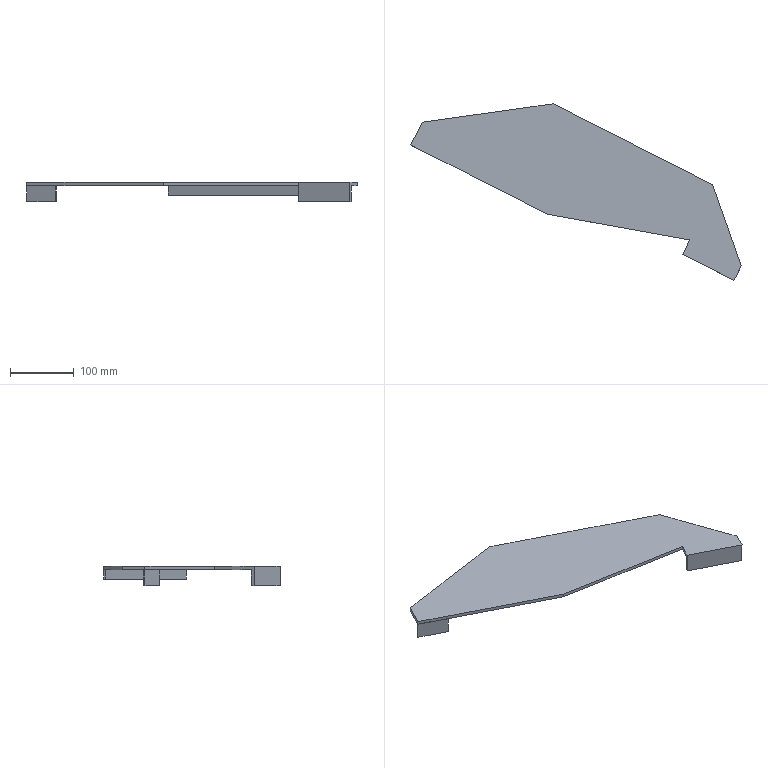Component | SolidWorks | Part17-1 | 2 solids | 23 faces | box 517.58 x 276.19 x 30 mm | volume 334372 mm3 | plane 23
build123d program:
from build123d import *

# Parameters (mm, degrees)
SKETCH1_W           = 90
SKETCH1_H           = 30
BOSS_EXTRUDE1_DEPTH = 5
BOSS_EXTRUDE2_DEPTH = 5
SKETCH3_W           = 280
SKETCH3_H           = 15
BOSS_EXTRUDE7_DEPTH = 3
BOSS_EXTRUDE8_DEPTH = 3


with BuildPart() as part:
    # Sketch1 → Boss-Extrude1 (new body)
    with BuildSketch(Plane.XY):
        with Locations((-7.063, 15)):
            Rectangle(SKETCH1_W, SKETCH1_H)
    extrude(amount=BOSS_EXTRUDE1_DEPTH)

    # Sketch2 → Boss-Extrude2 (add)
    with BuildSketch(Plane(origin=(0, 30, 0), x_dir=(-1, 0, 0), z_dir=(0, -1, 0))):
        Polygon((-37.937, 0), (-37.937, 20), (59.702, 113.229), (339.702, 113.229), (509.386, -5), (509.386, -45), (269.386, -45), (52.063, 20), (52.063, 0), (52.063, -5), (-37.937, -5), align=None)
    extrude(amount=BOSS_EXTRUDE2_DEPTH)

    # Sketch3 → Boss-Extrude7 (add)
    with BuildSketch(Plane(origin=(0, 0, -113.229), x_dir=(-1, 0, 0), z_dir=(0, 0, -1))):
        with Locations((199.702, 17.5)):
            Rectangle(SKETCH3_W, SKETCH3_H)
    extrude(amount=-BOSS_EXTRUDE7_DEPTH)


with BuildPart() as body_2:
    # Sketch6 → Boss-Extrude8 (new body)
    with BuildSketch(Plane.XY.offset(45)):
        Polygon((-509.386, 25), (-509.386, 0), (-459.386, 0), (-459.386, 24.804), align=None)
    extrude(amount=-BOSS_EXTRUDE8_DEPTH)


solid = Compound([part.part, body_2.part])

# Placed as in the assembly
solid = solid.moved(Location((298.812, -1061.476, 2432.971), (90, -26.879, 0)))
STEP:
#1=COLOUR_RGB('',0.7922,0.8196,0.9333);
#2=FILL_AREA_STYLE_COLOUR('',#1);
#3=FILL_AREA_STYLE('',(#2));
#4=SURFACE_STYLE_FILL_AREA(#3);
#5=SURFACE_SIDE_STYLE('',(#4));
#6=SURFACE_STYLE_USAGE(.BOTH.,#5);
#7=PRESENTATION_STYLE_ASSIGNMENT((#6));
#8=CARTESIAN_POINT('',(-6.213,-32.899,96.771));
#9=VERTEX_POINT('',#8);
#10=CARTESIAN_POINT('',(1.85,-31.768,96.771));
#11=VERTEX_POINT('',#10);
#12=CARTESIAN_POINT('',(-6.213,-32.899,96.771));
#13=DIRECTION('',(0.9903,0.139,0.));
#14=VECTOR('',#13,39.37);
#15=LINE('',#12,#14);
#16=EDGE_CURVE('',#9,#11,#15,.T.);
#17=ORIENTED_EDGE('',*,*,#16,.T.);
#18=CARTESIAN_POINT('',(1.797,-31.873,96.771));
#19=VERTEX_POINT('',#18);
#20=CARTESIAN_POINT('',(1.797,-31.873,96.771));
#21=DIRECTION('',(0.4521,0.892,0.));
#22=VECTOR('',#21,39.37);
#23=LINE('',#20,#22);
#24=EDGE_CURVE('',#19,#11,#23,.T.);
#25=ORIENTED_EDGE('',*,*,#24,.F.);
#26=CARTESIAN_POINT('',(11.63,-36.857,96.771));
#27=VERTEX_POINT('',#26);
#28=CARTESIAN_POINT('',(11.63,-36.857,96.771));
#29=DIRECTION('',(-0.892,0.4521,0.));
#30=VECTOR('',#29,39.37);
#31=LINE('',#28,#30);
#32=EDGE_CURVE('',#27,#19,#31,.T.);
#33=ORIENTED_EDGE('',*,*,#32,.F.);
#34=CARTESIAN_POINT('',(11.683,-36.751,96.771));
#35=VERTEX_POINT('',#34);
#36=CARTESIAN_POINT('',(11.63,-36.857,96.771));
#37=DIRECTION('',(0.4521,0.892,0.));
#38=VECTOR('',#37,39.37);
#39=LINE('',#36,#38);
#40=EDGE_CURVE('',#27,#35,#39,.T.);
#41=ORIENTED_EDGE('',*,*,#40,.T.);
#42=CARTESIAN_POINT('',(13.452,-41.763,96.771));
#43=VERTEX_POINT('',#42);
#44=CARTESIAN_POINT('',(13.452,-41.763,96.771));
#45=DIRECTION('',(0.3329,-0.943,-0.));
#46=VECTOR('',#45,39.37);
#47=LINE('',#44,#46);
#48=EDGE_CURVE('',#35,#43,#47,.T.);
#49=ORIENTED_EDGE('',*,*,#48,.T.);
#50=CARTESIAN_POINT('',(13.096,-42.466,96.771));
#51=VERTEX_POINT('',#50);
#52=CARTESIAN_POINT('',(13.096,-42.466,96.771));
#53=DIRECTION('',(-0.4521,-0.892,-0.));
#54=VECTOR('',#53,39.37);
#55=LINE('',#52,#54);
#56=EDGE_CURVE('',#43,#51,#55,.T.);
#57=ORIENTED_EDGE('',*,*,#56,.T.);
#58=CARTESIAN_POINT('',(9.936,-40.864,96.771));
#59=VERTEX_POINT('',#58);
#60=CARTESIAN_POINT('',(11.764,-41.79,96.771));
#61=DIRECTION('',(0.892,-0.4521,-0.));
#62=VECTOR('',#61,39.37);
#63=LINE('',#60,#62);
#64=EDGE_CURVE('',#59,#51,#63,.T.);
#65=ORIENTED_EDGE('',*,*,#64,.F.);
#66=CARTESIAN_POINT('',(10.292,-40.161,96.771));
#67=VERTEX_POINT('',#66);
#68=CARTESIAN_POINT('',(9.847,-41.039,96.771));
#69=DIRECTION('',(0.4521,0.892,0.));
#70=VECTOR('',#69,39.37);
#71=LINE('',#68,#70);
#72=EDGE_CURVE('',#59,#67,#71,.T.);
#73=ORIENTED_EDGE('',*,*,#72,.T.);
#74=CARTESIAN_POINT('',(1.503,-38.576,96.771));
#75=VERTEX_POINT('',#74);
#76=CARTESIAN_POINT('',(10.292,-40.161,96.771));
#77=DIRECTION('',(-0.9841,0.1775,0.));
#78=VECTOR('',#77,39.37);
#79=LINE('',#76,#78);
#80=EDGE_CURVE('',#67,#75,#79,.T.);
#81=ORIENTED_EDGE('',*,*,#80,.T.);
#82=CARTESIAN_POINT('',(-6.925,-34.304,96.771));
#83=VERTEX_POINT('',#82);
#84=CARTESIAN_POINT('',(1.503,-38.576,96.771));
#85=DIRECTION('',(-0.892,0.4521,0.));
#86=VECTOR('',#85,39.37);
#87=LINE('',#84,#86);
#88=EDGE_CURVE('',#75,#83,#87,.T.);
#89=ORIENTED_EDGE('',*,*,#88,.T.);
#90=CARTESIAN_POINT('',(-6.925,-34.304,96.771));
#91=DIRECTION('',(0.4521,0.892,0.));
#92=VECTOR('',#91,39.37);
#93=LINE('',#90,#92);
#94=EDGE_CURVE('',#83,#9,#93,.T.);
#95=ORIENTED_EDGE('',*,*,#94,.T.);
#96=EDGE_LOOP('',(#17,#25,#33,#41,#49,#57,#65,#73,#81,#89,#95));
#97=FACE_OUTER_BOUND('',#96,.T.);
#98=CARTESIAN_POINT('',(11.764,-41.79,96.771));
#99=DIRECTION('',(0.,0.,-1.));
#100=DIRECTION('',(0.4521,0.892,0.));
#101=AXIS2_PLACEMENT_3D('',#98,#99,#100);
#102=PLANE('',#101);
#103=ADVANCED_FACE('',(#97),#102,.T.);
#104=CARTESIAN_POINT('',(9.847,-41.039,95.786));
#105=VERTEX_POINT('',#104);
#106=CARTESIAN_POINT('',(9.936,-40.864,95.786));
#107=VERTEX_POINT('',#106);
#108=CARTESIAN_POINT('',(9.847,-41.039,95.786));
#109=DIRECTION('',(0.4521,0.892,0.));
#110=VECTOR('',#109,39.37);
#111=LINE('',#108,#110);
#112=EDGE_CURVE('',#105,#107,#111,.T.);
#113=ORIENTED_EDGE('',*,*,#112,.F.);
#114=CARTESIAN_POINT('',(9.847,-41.039,96.967));
#115=VERTEX_POINT('',#114);
#116=CARTESIAN_POINT('',(9.847,-41.039,96.967));
#117=DIRECTION('',(0.,0.,-1.));
#118=VECTOR('',#117,39.37);
#119=LINE('',#116,#118);
#120=EDGE_CURVE('',#115,#105,#119,.T.);
#121=ORIENTED_EDGE('',*,*,#120,.F.);
#122=CARTESIAN_POINT('',(10.292,-40.161,96.967));
#123=VERTEX_POINT('',#122);
#124=CARTESIAN_POINT('',(9.847,-41.039,96.967));
#125=DIRECTION('',(0.4521,0.892,0.));
#126=VECTOR('',#125,39.37);
#127=LINE('',#124,#126);
#128=EDGE_CURVE('',#115,#123,#127,.T.);
#129=ORIENTED_EDGE('',*,*,#128,.T.);
#130=CARTESIAN_POINT('',(10.292,-40.161,96.771));
#131=DIRECTION('',(-0.,-0.,1.));
#132=VECTOR('',#131,39.37);
#133=LINE('',#130,#132);
#134=EDGE_CURVE('',#67,#123,#133,.T.);
#135=ORIENTED_EDGE('',*,*,#134,.F.);
#136=ORIENTED_EDGE('',*,*,#72,.F.);
#137=CARTESIAN_POINT('',(9.936,-40.864,96.967));
#138=DIRECTION('',(0.,0.,-1.));
#139=VECTOR('',#138,39.37);
#140=LINE('',#137,#139);
#141=EDGE_CURVE('',#59,#107,#140,.T.);
#142=ORIENTED_EDGE('',*,*,#141,.T.);
#143=EDGE_LOOP('',(#113,#121,#129,#135,#136,#142));
#144=FACE_OUTER_BOUND('',#143,.T.);
#145=CARTESIAN_POINT('',(9.847,-41.039,96.967));
#146=DIRECTION('',(0.892,-0.4521,-0.));
#147=DIRECTION('',(0.4521,0.892,0.));
#148=AXIS2_PLACEMENT_3D('',#145,#146,#147);
#149=PLANE('',#148);
#150=ADVANCED_FACE('',(#144),#149,.F.);
#151=CARTESIAN_POINT('',(13.096,-42.466,95.786));
#152=VERTEX_POINT('',#151);
#153=CARTESIAN_POINT('',(9.936,-40.864,95.786));
#154=DIRECTION('',(0.892,-0.4521,-0.));
#155=VECTOR('',#154,39.37);
#156=LINE('',#153,#155);
#157=EDGE_CURVE('',#107,#152,#156,.T.);
#158=ORIENTED_EDGE('',*,*,#157,.T.);
#159=CARTESIAN_POINT('',(13.007,-42.641,95.786));
#160=VERTEX_POINT('',#159);
#161=CARTESIAN_POINT('',(13.007,-42.641,95.786));
#162=DIRECTION('',(0.4521,0.892,0.));
#163=VECTOR('',#162,39.37);
#164=LINE('',#161,#163);
#165=EDGE_CURVE('',#160,#152,#164,.T.);
#166=ORIENTED_EDGE('',*,*,#165,.F.);
#167=CARTESIAN_POINT('',(9.847,-41.039,95.786));
#168=DIRECTION('',(0.892,-0.4521,-0.));
#169=VECTOR('',#168,39.37);
#170=LINE('',#167,#169);
#171=EDGE_CURVE('',#105,#160,#170,.T.);
#172=ORIENTED_EDGE('',*,*,#171,.F.);
#173=ORIENTED_EDGE('',*,*,#112,.T.);
#174=EDGE_LOOP('',(#158,#166,#172,#173));
#175=FACE_OUTER_BOUND('',#174,.T.);
#176=CARTESIAN_POINT('',(9.847,-41.039,95.786));
#177=DIRECTION('',(-0.,-0.,1.));
#178=DIRECTION('',(-0.4521,-0.892,-0.));
#179=AXIS2_PLACEMENT_3D('',#176,#177,#178);
#180=PLANE('',#179);
#181=ADVANCED_FACE('',(#175),#180,.F.);
#182=CARTESIAN_POINT('',(13.096,-42.466,96.967));
#183=DIRECTION('',(-0.,-0.,1.));
#184=VECTOR('',#183,39.37);
#185=LINE('',#182,#184);
#186=EDGE_CURVE('',#152,#51,#185,.T.);
#187=ORIENTED_EDGE('',*,*,#186,.T.);
#188=ORIENTED_EDGE('',*,*,#56,.F.);
#189=CARTESIAN_POINT('',(13.452,-41.763,96.967));
#190=VERTEX_POINT('',#189);
#191=CARTESIAN_POINT('',(13.452,-41.763,96.771));
#192=DIRECTION('',(-0.,-0.,1.));
#193=VECTOR('',#192,39.37);
#194=LINE('',#191,#193);
#195=EDGE_CURVE('',#43,#190,#194,.T.);
#196=ORIENTED_EDGE('',*,*,#195,.T.);
#197=CARTESIAN_POINT('',(13.007,-42.641,96.967));
#198=VERTEX_POINT('',#197);
#199=CARTESIAN_POINT('',(13.007,-42.641,96.967));
#200=DIRECTION('',(0.4521,0.892,0.));
#201=VECTOR('',#200,39.37);
#202=LINE('',#199,#201);
#203=EDGE_CURVE('',#198,#190,#202,.T.);
#204=ORIENTED_EDGE('',*,*,#203,.F.);
#205=CARTESIAN_POINT('',(13.007,-42.641,96.967));
#206=DIRECTION('',(-0.,-0.,1.));
#207=VECTOR('',#206,39.37);
#208=LINE('',#205,#207);
#209=EDGE_CURVE('',#160,#198,#208,.T.);
#210=ORIENTED_EDGE('',*,*,#209,.F.);
#211=ORIENTED_EDGE('',*,*,#165,.T.);
#212=EDGE_LOOP('',(#187,#188,#196,#204,#210,#211));
#213=FACE_OUTER_BOUND('',#212,.T.);
#214=CARTESIAN_POINT('',(13.007,-42.641,96.967));
#215=DIRECTION('',(-0.892,0.4521,0.));
#216=DIRECTION('',(-0.4521,-0.892,-0.));
#217=AXIS2_PLACEMENT_3D('',#214,#215,#216);
#218=PLANE('',#217);
#219=ADVANCED_FACE('',(#213),#218,.F.);
#220=ORIENTED_EDGE('',*,*,#203,.T.);
#221=CARTESIAN_POINT('',(11.683,-36.751,96.967));
#222=VERTEX_POINT('',#221);
#223=CARTESIAN_POINT('',(13.452,-41.763,96.967));
#224=DIRECTION('',(0.3329,-0.943,-0.));
#225=VECTOR('',#224,39.37);
#226=LINE('',#223,#225);
#227=EDGE_CURVE('',#222,#190,#226,.T.);
#228=ORIENTED_EDGE('',*,*,#227,.F.);
#229=CARTESIAN_POINT('',(1.85,-31.768,96.967));
#230=VERTEX_POINT('',#229);
#231=CARTESIAN_POINT('',(11.683,-36.751,96.967));
#232=DIRECTION('',(0.892,-0.4521,-0.));
#233=VECTOR('',#232,39.37);
#234=LINE('',#231,#233);
#235=EDGE_CURVE('',#230,#222,#234,.T.);
#236=ORIENTED_EDGE('',*,*,#235,.F.);
#237=CARTESIAN_POINT('',(-6.213,-32.899,96.967));
#238=VERTEX_POINT('',#237);
#239=CARTESIAN_POINT('',(-6.213,-32.899,96.967));
#240=DIRECTION('',(0.9903,0.139,0.));
#241=VECTOR('',#240,39.37);
#242=LINE('',#239,#241);
#243=EDGE_CURVE('',#238,#230,#242,.T.);
#244=ORIENTED_EDGE('',*,*,#243,.F.);
#245=CARTESIAN_POINT('',(-6.925,-34.304,96.967));
#246=VERTEX_POINT('',#245);
#247=CARTESIAN_POINT('',(-6.925,-34.304,96.967));
#248=DIRECTION('',(0.4521,0.892,0.));
#249=VECTOR('',#248,39.37);
#250=LINE('',#247,#249);
#251=EDGE_CURVE('',#246,#238,#250,.T.);
#252=ORIENTED_EDGE('',*,*,#251,.F.);
#253=CARTESIAN_POINT('',(1.503,-38.576,96.967));
#254=VERTEX_POINT('',#253);
#255=CARTESIAN_POINT('',(1.503,-38.576,96.967));
#256=DIRECTION('',(-0.892,0.4521,0.));
#257=VECTOR('',#256,39.37);
#258=LINE('',#255,#257);
#259=EDGE_CURVE('',#254,#246,#258,.T.);
#260=ORIENTED_EDGE('',*,*,#259,.F.);
#261=CARTESIAN_POINT('',(10.292,-40.161,96.967));
#262=DIRECTION('',(-0.9841,0.1775,0.));
#263=VECTOR('',#262,39.37);
#264=LINE('',#261,#263);
#265=EDGE_CURVE('',#123,#254,#264,.T.);
#266=ORIENTED_EDGE('',*,*,#265,.F.);
#267=ORIENTED_EDGE('',*,*,#128,.F.);
#268=CARTESIAN_POINT('',(9.847,-41.039,96.967));
#269=DIRECTION('',(-0.892,0.4521,0.));
#270=VECTOR('',#269,39.37);
#271=LINE('',#268,#270);
#272=EDGE_CURVE('',#198,#115,#271,.T.);
#273=ORIENTED_EDGE('',*,*,#272,.F.);
#274=EDGE_LOOP('',(#220,#228,#236,#244,#252,#260,#266,#267,#273));
#275=FACE_OUTER_BOUND('',#274,.T.);
#276=CARTESIAN_POINT('',(9.847,-41.039,96.967));
#277=DIRECTION('',(0.,0.,-1.));
#278=DIRECTION('',(0.4521,0.892,0.));
#279=AXIS2_PLACEMENT_3D('',#276,#277,#278);
#280=PLANE('',#279);
#281=ADVANCED_FACE('',(#275),#280,.F.);
#282=ORIENTED_EDGE('',*,*,#209,.T.);
#283=ORIENTED_EDGE('',*,*,#272,.T.);
#284=ORIENTED_EDGE('',*,*,#120,.T.);
#285=ORIENTED_EDGE('',*,*,#171,.T.);
#286=EDGE_LOOP('',(#282,#283,#284,#285));
#287=FACE_OUTER_BOUND('',#286,.T.);
#288=CARTESIAN_POINT('',(11.675,-41.966,95.786));
#289=DIRECTION('',(-0.4521,-0.892,-0.));
#290=DIRECTION('',(0.892,-0.4521,-0.));
#291=AXIS2_PLACEMENT_3D('',#288,#289,#290);
#292=PLANE('',#291);
#293=ADVANCED_FACE('',(#287),#292,.T.);
#294=ORIENTED_EDGE('',*,*,#141,.F.);
#295=ORIENTED_EDGE('',*,*,#64,.T.);
#296=ORIENTED_EDGE('',*,*,#186,.F.);
#297=ORIENTED_EDGE('',*,*,#157,.F.);
#298=EDGE_LOOP('',(#294,#295,#296,#297));
#299=FACE_OUTER_BOUND('',#298,.T.);
#300=CARTESIAN_POINT('',(11.764,-41.79,95.786));
#301=DIRECTION('',(-0.4521,-0.892,-0.));
#302=DIRECTION('',(0.892,-0.4521,-0.));
#303=AXIS2_PLACEMENT_3D('',#300,#301,#302);
#304=PLANE('',#303);
#305=ADVANCED_FACE('',(#299),#304,.F.);
#306=ORIENTED_EDGE('',*,*,#265,.T.);
#307=CARTESIAN_POINT('',(1.503,-38.576,96.771));
#308=DIRECTION('',(-0.,-0.,1.));
#309=VECTOR('',#308,39.37);
#310=LINE('',#307,#309);
#311=EDGE_CURVE('',#75,#254,#310,.T.);
#312=ORIENTED_EDGE('',*,*,#311,.F.);
#313=ORIENTED_EDGE('',*,*,#80,.F.);
#314=ORIENTED_EDGE('',*,*,#134,.T.);
#315=EDGE_LOOP('',(#306,#312,#313,#314));
#316=FACE_OUTER_BOUND('',#315,.T.);
#317=CARTESIAN_POINT('',(10.292,-40.161,96.771));
#318=DIRECTION('',(0.1775,0.9841,0.));
#319=DIRECTION('',(-0.9841,0.1775,0.));
#320=AXIS2_PLACEMENT_3D('',#317,#318,#319);
#321=PLANE('',#320);
#322=ADVANCED_FACE('',(#316),#321,.F.);
#323=ORIENTED_EDGE('',*,*,#259,.T.);
#324=CARTESIAN_POINT('',(-6.925,-34.304,96.771));
#325=DIRECTION('',(-0.,-0.,1.));
#326=VECTOR('',#325,39.37);
#327=LINE('',#324,#326);
#328=EDGE_CURVE('',#83,#246,#327,.T.);
#329=ORIENTED_EDGE('',*,*,#328,.F.);
#330=ORIENTED_EDGE('',*,*,#88,.F.);
#331=ORIENTED_EDGE('',*,*,#311,.T.);
#332=EDGE_LOOP('',(#323,#329,#330,#331));
#333=FACE_OUTER_BOUND('',#332,.T.);
#334=CARTESIAN_POINT('',(1.503,-38.576,96.771));
#335=DIRECTION('',(0.4521,0.892,0.));
#336=DIRECTION('',(-0.892,0.4521,0.));
#337=AXIS2_PLACEMENT_3D('',#334,#335,#336);
#338=PLANE('',#337);
#339=ADVANCED_FACE('',(#333),#338,.F.);
#340=ORIENTED_EDGE('',*,*,#251,.T.);
#341=CARTESIAN_POINT('',(-6.213,-32.899,96.771));
#342=DIRECTION('',(-0.,-0.,1.));
#343=VECTOR('',#342,39.37);
#344=LINE('',#341,#343);
#345=EDGE_CURVE('',#9,#238,#344,.T.);
#346=ORIENTED_EDGE('',*,*,#345,.F.);
#347=ORIENTED_EDGE('',*,*,#94,.F.);
#348=ORIENTED_EDGE('',*,*,#328,.T.);
#349=EDGE_LOOP('',(#340,#346,#347,#348));
#350=FACE_OUTER_BOUND('',#349,.T.);
#351=CARTESIAN_POINT('',(-6.925,-34.304,96.771));
#352=DIRECTION('',(0.892,-0.4521,-0.));
#353=DIRECTION('',(0.4521,0.892,0.));
#354=AXIS2_PLACEMENT_3D('',#351,#352,#353);
#355=PLANE('',#354);
#356=ADVANCED_FACE('',(#350),#355,.F.);
#357=ORIENTED_EDGE('',*,*,#243,.T.);
#358=CARTESIAN_POINT('',(1.85,-31.768,96.771));
#359=DIRECTION('',(-0.,-0.,1.));
#360=VECTOR('',#359,39.37);
#361=LINE('',#358,#360);
#362=EDGE_CURVE('',#11,#230,#361,.T.);
#363=ORIENTED_EDGE('',*,*,#362,.F.);
#364=ORIENTED_EDGE('',*,*,#16,.F.);
#365=ORIENTED_EDGE('',*,*,#345,.T.);
#366=EDGE_LOOP('',(#357,#363,#364,#365));
#367=FACE_OUTER_BOUND('',#366,.T.);
#368=CARTESIAN_POINT('',(-6.213,-32.899,96.771));
#369=DIRECTION('',(0.139,-0.9903,-0.));
#370=DIRECTION('',(0.9903,0.139,0.));
#371=AXIS2_PLACEMENT_3D('',#368,#369,#370);
#372=PLANE('',#371);
#373=ADVANCED_FACE('',(#367),#372,.F.);
#374=ORIENTED_EDGE('',*,*,#235,.T.);
#375=CARTESIAN_POINT('',(11.683,-36.751,96.771));
#376=DIRECTION('',(-0.,-0.,1.));
#377=VECTOR('',#376,39.37);
#378=LINE('',#375,#377);
#379=EDGE_CURVE('',#35,#222,#378,.T.);
#380=ORIENTED_EDGE('',*,*,#379,.F.);
#381=CARTESIAN_POINT('',(11.683,-36.751,96.18));
#382=VERTEX_POINT('',#381);
#383=CARTESIAN_POINT('',(11.683,-36.751,96.771));
#384=DIRECTION('',(0.,0.,-1.));
#385=VECTOR('',#384,39.37);
#386=LINE('',#383,#385);
#387=EDGE_CURVE('',#35,#382,#386,.T.);
#388=ORIENTED_EDGE('',*,*,#387,.T.);
#389=CARTESIAN_POINT('',(1.85,-31.768,96.18));
#390=VERTEX_POINT('',#389);
#391=CARTESIAN_POINT('',(11.683,-36.751,96.18));
#392=DIRECTION('',(-0.892,0.4521,0.));
#393=VECTOR('',#392,39.37);
#394=LINE('',#391,#393);
#395=EDGE_CURVE('',#382,#390,#394,.T.);
#396=ORIENTED_EDGE('',*,*,#395,.T.);
#397=CARTESIAN_POINT('',(1.85,-31.768,96.771));
#398=DIRECTION('',(0.,0.,-1.));
#399=VECTOR('',#398,39.37);
#400=LINE('',#397,#399);
#401=EDGE_CURVE('',#11,#390,#400,.T.);
#402=ORIENTED_EDGE('',*,*,#401,.F.);
#403=ORIENTED_EDGE('',*,*,#362,.T.);
#404=EDGE_LOOP('',(#374,#380,#388,#396,#402,#403));
#405=FACE_OUTER_BOUND('',#404,.T.);
#406=CARTESIAN_POINT('',(11.683,-36.751,96.771));
#407=DIRECTION('',(-0.4521,-0.892,-0.));
#408=DIRECTION('',(0.892,-0.4521,-0.));
#409=AXIS2_PLACEMENT_3D('',#406,#407,#408);
#410=PLANE('',#409);
#411=ADVANCED_FACE('',(#405),#410,.F.);
#412=ORIENTED_EDGE('',*,*,#227,.T.);
#413=ORIENTED_EDGE('',*,*,#195,.F.);
#414=ORIENTED_EDGE('',*,*,#48,.F.);
#415=ORIENTED_EDGE('',*,*,#379,.T.);
#416=EDGE_LOOP('',(#412,#413,#414,#415));
#417=FACE_OUTER_BOUND('',#416,.T.);
#418=CARTESIAN_POINT('',(13.452,-41.763,96.771));
#419=DIRECTION('',(-0.943,-0.3329,-0.));
#420=DIRECTION('',(0.3329,-0.943,-0.));
#421=AXIS2_PLACEMENT_3D('',#418,#419,#420);
#422=PLANE('',#421);
#423=ADVANCED_FACE('',(#417),#422,.F.);
#424=ORIENTED_EDGE('',*,*,#401,.T.);
#425=CARTESIAN_POINT('',(1.797,-31.873,96.18));
#426=VERTEX_POINT('',#425);
#427=CARTESIAN_POINT('',(1.797,-31.873,96.18));
#428=DIRECTION('',(0.4521,0.892,0.));
#429=VECTOR('',#428,39.37);
#430=LINE('',#427,#429);
#431=EDGE_CURVE('',#426,#390,#430,.T.);
#432=ORIENTED_EDGE('',*,*,#431,.F.);
#433=CARTESIAN_POINT('',(1.797,-31.873,96.771));
#434=DIRECTION('',(0.,0.,-1.));
#435=VECTOR('',#434,39.37);
#436=LINE('',#433,#435);
#437=EDGE_CURVE('',#19,#426,#436,.T.);
#438=ORIENTED_EDGE('',*,*,#437,.F.);
#439=ORIENTED_EDGE('',*,*,#24,.T.);
#440=EDGE_LOOP('',(#424,#432,#438,#439));
#441=FACE_OUTER_BOUND('',#440,.T.);
#442=CARTESIAN_POINT('',(1.797,-31.873,96.771));
#443=DIRECTION('',(0.892,-0.4521,-0.));
#444=DIRECTION('',(0.4521,0.892,0.));
#445=AXIS2_PLACEMENT_3D('',#442,#443,#444);
#446=PLANE('',#445);
#447=ADVANCED_FACE('',(#441),#446,.F.);
#448=ORIENTED_EDGE('',*,*,#395,.F.);
#449=CARTESIAN_POINT('',(11.63,-36.857,96.18));
#450=VERTEX_POINT('',#449);
#451=CARTESIAN_POINT('',(11.63,-36.857,96.18));
#452=DIRECTION('',(0.4521,0.892,0.));
#453=VECTOR('',#452,39.37);
#454=LINE('',#451,#453);
#455=EDGE_CURVE('',#450,#382,#454,.T.);
#456=ORIENTED_EDGE('',*,*,#455,.F.);
#457=CARTESIAN_POINT('',(11.63,-36.857,96.18));
#458=DIRECTION('',(-0.892,0.4521,0.));
#459=VECTOR('',#458,39.37);
#460=LINE('',#457,#459);
#461=EDGE_CURVE('',#450,#426,#460,.T.);
#462=ORIENTED_EDGE('',*,*,#461,.T.);
#463=ORIENTED_EDGE('',*,*,#431,.T.);
#464=EDGE_LOOP('',(#448,#456,#462,#463));
#465=FACE_OUTER_BOUND('',#464,.T.);
#466=CARTESIAN_POINT('',(11.63,-36.857,96.18));
#467=DIRECTION('',(0.,0.,-1.));
#468=DIRECTION('',(0.4521,0.892,0.));
#469=AXIS2_PLACEMENT_3D('',#466,#467,#468);
#470=PLANE('',#469);
#471=ADVANCED_FACE('',(#465),#470,.T.);
#472=ORIENTED_EDGE('',*,*,#387,.F.);
#473=ORIENTED_EDGE('',*,*,#40,.F.);
#474=CARTESIAN_POINT('',(11.63,-36.857,96.771));
#475=DIRECTION('',(0.,0.,-1.));
#476=VECTOR('',#475,39.37);
#477=LINE('',#474,#476);
#478=EDGE_CURVE('',#27,#450,#477,.T.);
#479=ORIENTED_EDGE('',*,*,#478,.T.);
#480=ORIENTED_EDGE('',*,*,#455,.T.);
#481=EDGE_LOOP('',(#472,#473,#479,#480));
#482=FACE_OUTER_BOUND('',#481,.T.);
#483=CARTESIAN_POINT('',(11.63,-36.857,96.771));
#484=DIRECTION('',(0.892,-0.4521,-0.));
#485=DIRECTION('',(0.4521,0.892,0.));
#486=AXIS2_PLACEMENT_3D('',#483,#484,#485);
#487=PLANE('',#486);
#488=ADVANCED_FACE('',(#482),#487,.T.);
#489=ORIENTED_EDGE('',*,*,#437,.T.);
#490=ORIENTED_EDGE('',*,*,#461,.F.);
#491=ORIENTED_EDGE('',*,*,#478,.F.);
#492=ORIENTED_EDGE('',*,*,#32,.T.);
#493=EDGE_LOOP('',(#489,#490,#491,#492));
#494=FACE_OUTER_BOUND('',#493,.T.);
#495=CARTESIAN_POINT('',(13.726,-37.919,95.786));
#496=DIRECTION('',(0.4521,0.892,0.));
#497=DIRECTION('',(-0.892,0.4521,0.));
#498=AXIS2_PLACEMENT_3D('',#495,#496,#497);
#499=PLANE('',#498);
#500=ADVANCED_FACE('',(#494),#499,.F.);
#501=CLOSED_SHELL('',(#103,#150,#181,#219,#281,#293,#305,#322,#339,#356,#373,#411,#423,#447,#471,#488,#500));
#502=MANIFOLD_SOLID_BREP('',#501);
#503=STYLED_ITEM('',(#7),#502);
#504=(LENGTH_UNIT()NAMED_UNIT(*)SI_UNIT($,.METRE.));
#505=LENGTH_MEASURE_WITH_UNIT(LENGTH_MEASURE(0.0254),#504);
#506=DIMENSIONAL_EXPONENTS(1.,0.,0.,0.,0.,0.,0.);
#507=(CONVERSION_BASED_UNIT('',#505)LENGTH_UNIT()NAMED_UNIT(#506));
#508=UNCERTAINTY_MEASURE_WITH_UNIT(LENGTH_MEASURE(0.00001),#507,'','');
#509=(NAMED_UNIT(*)PLANE_ANGLE_UNIT()SI_UNIT($,.RADIAN.));
#510=(NAMED_UNIT(*)SI_UNIT($,.STERADIAN.)SOLID_ANGLE_UNIT());
#511=(GEOMETRIC_REPRESENTATION_CONTEXT(3)GLOBAL_UNCERTAINTY_ASSIGNED_CONTEXT((#508))GLOBAL_UNIT_ASSIGNED_CONTEXT((#507,#509,#510))REPRESENTATION_CONTEXT('',''));
#512=MECHANICAL_DESIGN_GEOMETRIC_PRESENTATION_REPRESENTATION('',(#503),#511);
#513=COLOUR_RGB('',0.7922,0.8196,0.9333);
#514=FILL_AREA_STYLE_COLOUR('',#513);
#515=FILL_AREA_STYLE('',(#514));
#516=SURFACE_STYLE_FILL_AREA(#515);
#517=SURFACE_SIDE_STYLE('',(#516));
#518=SURFACE_STYLE_USAGE(.BOTH.,#517);
#519=PRESENTATION_STYLE_ASSIGNMENT((#518));
#520=CARTESIAN_POINT('',(-5.169,-35.194,96.763));
#521=VERTEX_POINT('',#520);
#522=CARTESIAN_POINT('',(-6.925,-34.304,96.771));
#523=VERTEX_POINT('',#522);
#524=CARTESIAN_POINT('',(-5.169,-35.194,96.763));
#525=DIRECTION('',(-0.892,0.4521,0.003912));
#526=VECTOR('',#525,39.37);
#527=LINE('',#524,#526);
#528=EDGE_CURVE('',#521,#523,#527,.T.);
#529=ORIENTED_EDGE('',*,*,#528,.F.);
#530=CARTESIAN_POINT('',(-5.115,-35.089,96.763));
#531=VERTEX_POINT('',#530);
#532=CARTESIAN_POINT('',(-5.115,-35.089,96.763));
#533=DIRECTION('',(-0.4521,-0.892,-0.));
#534=VECTOR('',#533,39.37);
#535=LINE('',#532,#534);
#536=EDGE_CURVE('',#531,#521,#535,.T.);
#537=ORIENTED_EDGE('',*,*,#536,.F.);
#538=CARTESIAN_POINT('',(-6.871,-34.199,96.771));
#539=VERTEX_POINT('',#538);
#540=CARTESIAN_POINT('',(-5.115,-35.089,96.763));
#541=DIRECTION('',(-0.892,0.4521,0.003912));
#542=VECTOR('',#541,39.37);
#543=LINE('',#540,#542);
#544=EDGE_CURVE('',#531,#539,#543,.T.);
#545=ORIENTED_EDGE('',*,*,#544,.T.);
#546=CARTESIAN_POINT('',(-6.871,-34.199,96.771));
#547=DIRECTION('',(-0.4521,-0.892,-0.));
#548=VECTOR('',#547,39.37);
#549=LINE('',#546,#548);
#550=EDGE_CURVE('',#539,#523,#549,.T.);
#551=ORIENTED_EDGE('',*,*,#550,.T.);
#552=EDGE_LOOP('',(#529,#537,#545,#551));
#553=FACE_OUTER_BOUND('',#552,.T.);
#554=CARTESIAN_POINT('',(-5.115,-35.089,96.763));
#555=DIRECTION('',(0.003489,-0.001769,1.));
#556=DIRECTION('',(-0.892,0.4521,0.003912));
#557=AXIS2_PLACEMENT_3D('',#554,#555,#556);
#558=PLANE('',#557);
#559=ADVANCED_FACE('',(#553),#558,.T.);
#560=CARTESIAN_POINT('',(-5.169,-35.194,95.786));
#561=VERTEX_POINT('',#560);
#562=CARTESIAN_POINT('',(-5.169,-35.194,95.786));
#563=DIRECTION('',(-0.,-0.,1.));
#564=VECTOR('',#563,39.37);
#565=LINE('',#562,#564);
#566=EDGE_CURVE('',#561,#521,#565,.T.);
#567=ORIENTED_EDGE('',*,*,#566,.F.);
#568=CARTESIAN_POINT('',(-5.115,-35.089,95.786));
#569=VERTEX_POINT('',#568);
#570=CARTESIAN_POINT('',(-5.115,-35.089,95.786));
#571=DIRECTION('',(-0.4521,-0.892,-0.));
#572=VECTOR('',#571,39.37);
#573=LINE('',#570,#572);
#574=EDGE_CURVE('',#569,#561,#573,.T.);
#575=ORIENTED_EDGE('',*,*,#574,.F.);
#576=CARTESIAN_POINT('',(-5.115,-35.089,95.786));
#577=DIRECTION('',(-0.,-0.,1.));
#578=VECTOR('',#577,39.37);
#579=LINE('',#576,#578);
#580=EDGE_CURVE('',#569,#531,#579,.T.);
#581=ORIENTED_EDGE('',*,*,#580,.T.);
#582=ORIENTED_EDGE('',*,*,#536,.T.);
#583=EDGE_LOOP('',(#567,#575,#581,#582));
#584=FACE_OUTER_BOUND('',#583,.T.);
#585=CARTESIAN_POINT('',(-5.115,-35.089,95.786));
#586=DIRECTION('',(0.892,-0.4521,-0.));
#587=DIRECTION('',(0.4521,0.892,0.));
#588=AXIS2_PLACEMENT_3D('',#585,#586,#587);
#589=PLANE('',#588);
#590=ADVANCED_FACE('',(#584),#589,.T.);
#591=CARTESIAN_POINT('',(-6.925,-34.304,95.786));
#592=VERTEX_POINT('',#591);
#593=CARTESIAN_POINT('',(-6.925,-34.304,95.786));
#594=DIRECTION('',(0.892,-0.4521,-0.));
#595=VECTOR('',#594,39.37);
#596=LINE('',#593,#595);
#597=EDGE_CURVE('',#592,#561,#596,.T.);
#598=ORIENTED_EDGE('',*,*,#597,.F.);
#599=CARTESIAN_POINT('',(-6.871,-34.199,95.786));
#600=VERTEX_POINT('',#599);
#601=CARTESIAN_POINT('',(-6.871,-34.199,95.786));
#602=DIRECTION('',(-0.4521,-0.892,-0.));
#603=VECTOR('',#602,39.37);
#604=LINE('',#601,#603);
#605=EDGE_CURVE('',#600,#592,#604,.T.);
#606=ORIENTED_EDGE('',*,*,#605,.F.);
#607=CARTESIAN_POINT('',(-6.871,-34.199,95.786));
#608=DIRECTION('',(0.892,-0.4521,-0.));
#609=VECTOR('',#608,39.37);
#610=LINE('',#607,#609);
#611=EDGE_CURVE('',#600,#569,#610,.T.);
#612=ORIENTED_EDGE('',*,*,#611,.T.);
#613=ORIENTED_EDGE('',*,*,#574,.T.);
#614=EDGE_LOOP('',(#598,#606,#612,#613));
#615=FACE_OUTER_BOUND('',#614,.T.);
#616=CARTESIAN_POINT('',(-6.871,-34.199,95.786));
#617=DIRECTION('',(0.,0.,-1.));
#618=DIRECTION('',(0.892,-0.4521,-0.));
#619=AXIS2_PLACEMENT_3D('',#616,#617,#618);
#620=PLANE('',#619);
#621=ADVANCED_FACE('',(#615),#620,.T.);
#622=CARTESIAN_POINT('',(-6.925,-34.304,96.771));
#623=DIRECTION('',(0.,0.,-1.));
#624=VECTOR('',#623,39.37);
#625=LINE('',#622,#624);
#626=EDGE_CURVE('',#523,#592,#625,.T.);
#627=ORIENTED_EDGE('',*,*,#626,.F.);
#628=ORIENTED_EDGE('',*,*,#550,.F.);
#629=CARTESIAN_POINT('',(-6.871,-34.199,96.771));
#630=DIRECTION('',(0.,0.,-1.));
#631=VECTOR('',#630,39.37);
#632=LINE('',#629,#631);
#633=EDGE_CURVE('',#539,#600,#632,.T.);
#634=ORIENTED_EDGE('',*,*,#633,.T.);
#635=ORIENTED_EDGE('',*,*,#605,.T.);
#636=EDGE_LOOP('',(#627,#628,#634,#635));
#637=FACE_OUTER_BOUND('',#636,.T.);
#638=CARTESIAN_POINT('',(-6.871,-34.199,96.771));
#639=DIRECTION('',(-0.892,0.4521,0.));
#640=DIRECTION('',(-0.4521,-0.892,-0.));
#641=AXIS2_PLACEMENT_3D('',#638,#639,#640);
#642=PLANE('',#641);
#643=ADVANCED_FACE('',(#637),#642,.T.);
#644=ORIENTED_EDGE('',*,*,#544,.F.);
#645=ORIENTED_EDGE('',*,*,#580,.F.);
#646=ORIENTED_EDGE('',*,*,#611,.F.);
#647=ORIENTED_EDGE('',*,*,#633,.F.);
#648=EDGE_LOOP('',(#644,#645,#646,#647));
#649=FACE_OUTER_BOUND('',#648,.T.);
#650=CARTESIAN_POINT('',(11.017,-43.265,95.786));
#651=DIRECTION('',(-0.4521,-0.892,-0.));
#652=DIRECTION('',(0.892,-0.4521,-0.));
#653=AXIS2_PLACEMENT_3D('',#650,#651,#652);
#654=PLANE('',#653);
#655=ADVANCED_FACE('',(#649),#654,.F.);
#656=ORIENTED_EDGE('',*,*,#528,.T.);
#657=ORIENTED_EDGE('',*,*,#626,.T.);
#658=ORIENTED_EDGE('',*,*,#597,.T.);
#659=ORIENTED_EDGE('',*,*,#566,.T.);
#660=EDGE_LOOP('',(#656,#657,#658,#659));
#661=FACE_OUTER_BOUND('',#660,.T.);
#662=CARTESIAN_POINT('',(10.963,-43.371,95.786));
#663=DIRECTION('',(-0.4521,-0.892,-0.));
#664=DIRECTION('',(0.892,-0.4521,-0.));
#665=AXIS2_PLACEMENT_3D('',#662,#663,#664);
#666=PLANE('',#665);
#667=ADVANCED_FACE('',(#661),#666,.T.);
#668=CLOSED_SHELL('',(#559,#590,#621,#643,#655,#667));
#669=MANIFOLD_SOLID_BREP('',#668);
#670=STYLED_ITEM('',(#519),#669);
#671=PRESENTATION_LAYER_ASSIGNMENT('','',(#670));
#672=CARTESIAN_POINT('',(0.,0.,0.));
#673=DIRECTION('',(0.,0.,1.));
#674=DIRECTION('',(1.,0.,0.));
#675=AXIS2_PLACEMENT_3D('',#672,#673,#674);
#676=(LENGTH_UNIT()NAMED_UNIT(*)SI_UNIT($,.METRE.));
#677=LENGTH_MEASURE_WITH_UNIT(LENGTH_MEASURE(0.0254),#676);
#678=DIMENSIONAL_EXPONENTS(1.,0.,0.,0.,0.,0.,0.);
#679=(CONVERSION_BASED_UNIT('',#677)LENGTH_UNIT()NAMED_UNIT(#678));
#680=UNCERTAINTY_MEASURE_WITH_UNIT(LENGTH_MEASURE(0.00001),#679,'','');
#681=(NAMED_UNIT(*)PLANE_ANGLE_UNIT()SI_UNIT($,.RADIAN.));
#682=(NAMED_UNIT(*)SI_UNIT($,.STERADIAN.)SOLID_ANGLE_UNIT());
#683=(GEOMETRIC_REPRESENTATION_CONTEXT(3)GLOBAL_UNCERTAINTY_ASSIGNED_CONTEXT((#680))GLOBAL_UNIT_ASSIGNED_CONTEXT((#679,#681,#682))REPRESENTATION_CONTEXT('',''));
#684=ADVANCED_BREP_SHAPE_REPRESENTATION('',(#669,#502,#675),#683);
#685=PRESENTATION_LAYER_ASSIGNMENT('','',(#503));
#686=(LENGTH_UNIT()NAMED_UNIT(*)SI_UNIT($,.METRE.));
#687=LENGTH_MEASURE_WITH_UNIT(LENGTH_MEASURE(0.0254),#686);
#688=DIMENSIONAL_EXPONENTS(1.,0.,0.,0.,0.,0.,0.);
#689=(CONVERSION_BASED_UNIT('',#687)LENGTH_UNIT()NAMED_UNIT(#688));
#690=UNCERTAINTY_MEASURE_WITH_UNIT(LENGTH_MEASURE(0.00001),#689,'','');
#691=(NAMED_UNIT(*)PLANE_ANGLE_UNIT()SI_UNIT($,.RADIAN.));
#692=(NAMED_UNIT(*)SI_UNIT($,.STERADIAN.)SOLID_ANGLE_UNIT());
#693=(GEOMETRIC_REPRESENTATION_CONTEXT(3)GLOBAL_UNCERTAINTY_ASSIGNED_CONTEXT((#690))GLOBAL_UNIT_ASSIGNED_CONTEXT((#689,#691,#692))REPRESENTATION_CONTEXT('',''));
#694=MECHANICAL_DESIGN_GEOMETRIC_PRESENTATION_REPRESENTATION('',(#670),#693);